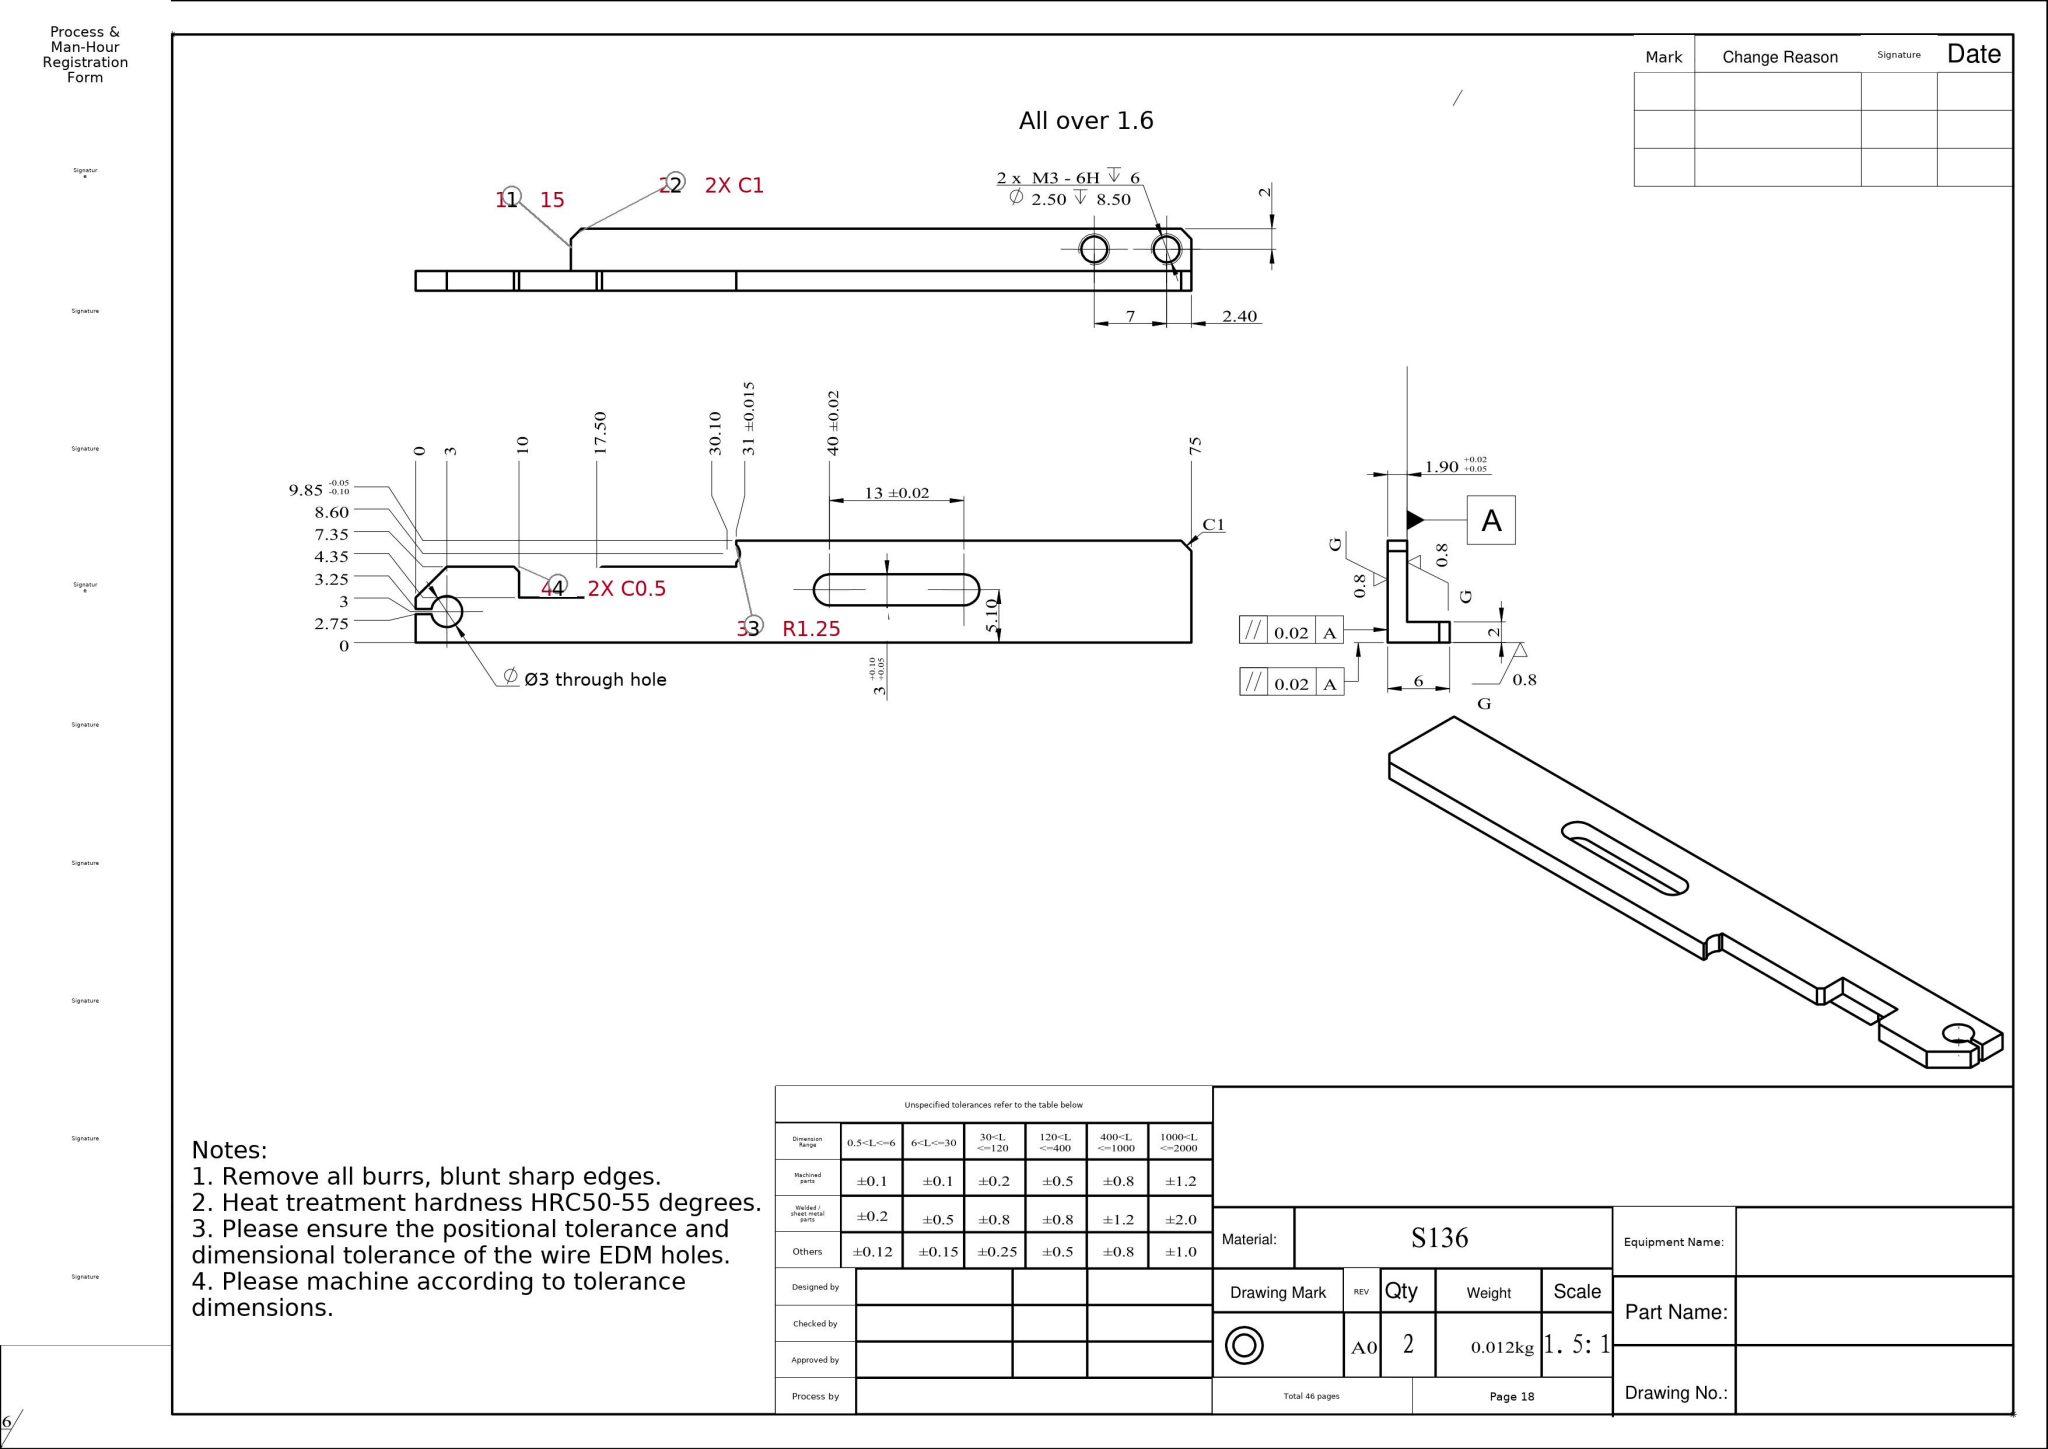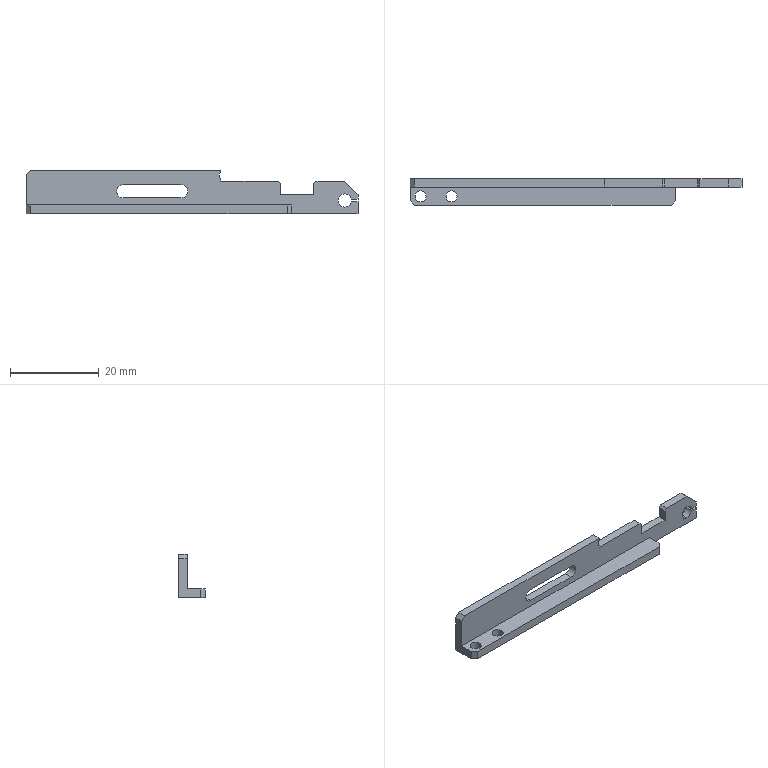Part | SolidWorks | mm | material S136 | 1 solid | 37 faces | box 75 x 6 x 9.85 mm | volume 1571 mm3 | plane 27 | cylinder 10 | commonest cylinder face diameters 2.5 x5 3 x5
build123d program:
from build123d import *

# Parameters (mm, degrees)
SKETCH1_W             = 75
SKETCH1_H             = 9.85
BOSS_EXTRUDE1_DEPTH   = 1.9
CUT_EXTRUDE2_DEPTH    = 76.668
SKETCH5_R             = 1.5
SKETCH5_W             = 6
SKETCH5_H             = 0.5
CUT_EXTRUDE3_DEPTH    = 1.9
CHAMFER1_SIZE         = 3
SKETCH6_R             = 1.25
CUT_EXTRUDE4_DEPTH    = 10
SKETCH8_W             = 60
SKETCH8_H             = 2
BOSS_EXTRUDE3_DEPTH   = 6
CHAMFER5_SIZE         = 1
CHAMFER6_SIZE         = 1
CHAMFER7_SIZE         = 0.5
M3_TAPPED_HOLE1_D     = 2.5
M3_TAPPED_HOLE1_DEPTH = 8.5
M3_TAPPED_HOLE1_TIP   = 0.7511


with BuildPart() as part:
    # Sketch1 → Boss-Extrude1 (new body)
    with BuildSketch(Plane(origin=(0, 0, 0), x_dir=(1, 0, 0), z_dir=(0, 1, 0))):
        with Locations((-37.5, -4.925)):
            Rectangle(SKETCH1_W, SKETCH1_H)
    extrude(amount=BOSS_EXTRUDE1_DEPTH)

    # Sketch4 → Cut-Extrude2 (cut, through all)
    with BuildSketch(Plane(origin=(0, 1.9, 0), x_dir=(1, 0, 0), z_dir=(0, 1, 0))):
        with BuildLine():
            Line((-53, -3.6), (-40, -3.6))
            ThreePointArc((-40, -3.6), (-38.5, -5.1), (-40, -6.6))
            Line((-40, -6.6), (-53, -6.6))
            ThreePointArc((-53, -6.6), (-54.5, -5.1), (-53, -3.6))
        make_face()
    extrude(amount=-CUT_EXTRUDE2_DEPTH, mode=Mode.SUBTRACT)

    # Sketch5 → Cut-Extrude3 (cut)
    with BuildSketch(Plane(origin=(0, 1.9, 0), x_dir=(1, 0, 0), z_dir=(0, 1, 0))):
        with Locations((-3, -3)):
            Circle(SKETCH5_R)
        with Locations((0, -3)):
            Rectangle(SKETCH5_W, SKETCH5_H)
        Polygon((-31, -9.85), (0, -9.85), (0, -7.35), (-10, -7.35), (-10, -4.35), (-17.5, -4.35), (-17.5, -7.35), (-31, -7.35), align=None)
    extrude(amount=-CUT_EXTRUDE3_DEPTH, mode=Mode.SUBTRACT)

    # Chamfer1
    chamfer1_edges = [part.edges().sort_by_distance(p)[0] for p in [
        (0, 0.95, 7.35),
    ]]
    chamfer(chamfer1_edges, length=CHAMFER1_SIZE)

    # Sketch6 → Cut-Extrude4 (cut)
    with BuildSketch(Plane(origin=(0, 1.9, 0), x_dir=(1, 0, 0), z_dir=(0, 1, 0))):
        with Locations((-30.1, -8.6)):
            Circle(SKETCH6_R)
    extrude(amount=-CUT_EXTRUDE4_DEPTH, mode=Mode.SUBTRACT)

    # Sketch8 → Boss-Extrude3 (add)
    with BuildSketch(Plane.XZ.offset(-1.9)):
        with Locations((-45, 1)):
            Rectangle(SKETCH8_W, SKETCH8_H)
    extrude(amount=BOSS_EXTRUDE3_DEPTH)

    # Chamfer5
    chamfer5_edges = [part.edges().sort_by_distance(p)[0] for p in [
        (-75, 0.95, 9.85),
    ]]
    chamfer(chamfer5_edges, length=CHAMFER5_SIZE)

    # Chamfer6
    chamfer6_edges = [part.edges().sort_by_distance(p)[0] for p in [
        (-75, -4.1, 1),
        (-15, -4.1, 1),
    ]]
    chamfer(chamfer6_edges, length=CHAMFER6_SIZE)

    # Chamfer7
    chamfer7_edges = [part.edges().sort_by_distance(p)[0] for p in [
        (-17.5, 0.95, 7.35),
        (-10, 0.95, 7.35),
    ]]
    chamfer(chamfer7_edges, length=CHAMFER7_SIZE)

    # M3 Tapped Hole1
    with Locations(Plane(origin=(0, 0, 0), x_dir=(-1, 0, 0), z_dir=(0, 0, -1))):
        with Locations((72.6, -2.1), (65.6, -2.1)):
            Hole(M3_TAPPED_HOLE1_D / 2, depth=M3_TAPPED_HOLE1_DEPTH)
            with Locations((0, 0, -(M3_TAPPED_HOLE1_DEPTH + M3_TAPPED_HOLE1_TIP / 2))):  # 118° drill point
                Cone(0, M3_TAPPED_HOLE1_D / 2, M3_TAPPED_HOLE1_TIP, mode=Mode.SUBTRACT)


solid = part.part